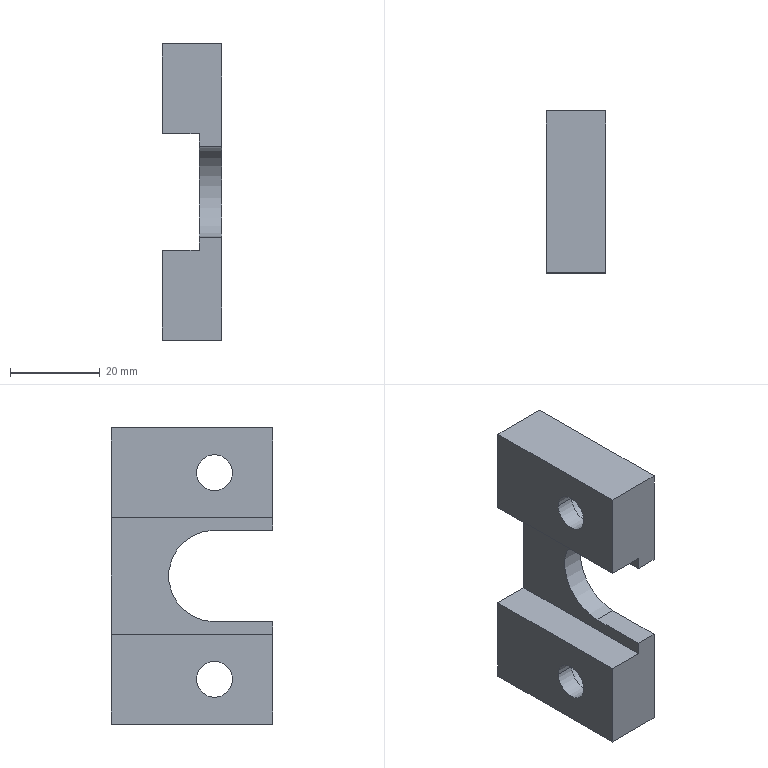Component | SolidWorks | ST60-12-1 | 1 solid | 24 faces | box 13.2 x 36 x 66 mm | volume 17942 mm3 | plane 15 | cylinder 9 | commonest cylinder face diameters 15 x4 8 x4 20.4 x1
build123d program:
from build123d import *

# Parameters (mm, degrees)
BOSS_EXTRUDE1_DEPTH                                = 46
CUT_EXTRUDE1_DEPTH                                 = 59.931
HOLE_SIZE_ACCORDING_TO_TYPE_1_OF_HEXAG_D           = 8
HOLE_SIZE_ACCORDING_TO_TYPE_1_OF_HEXAG_CBORE_D     = 15
HOLE_SIZE_ACCORDING_TO_TYPE_1_OF_HEXAG_CBORE_DEPTH = 9
SKETCH5_W                                          = 85.429
SKETCH5_H                                          = 31.164
CUT_EXTRUDE2_DEPTH                                 = 10


with BuildPart() as part:
    # Sketch1 → Boss-Extrude1 (new body)
    with BuildSketch(Plane.XY):
        Polygon((14.39, -6.081), (34.39, -6.081), (34.39, 7.119), (-31.61, 7.119), (-31.61, -6.081), (-11.61, -6.081), (-11.61, 2.119), (14.39, 2.119), align=None)
    extrude(amount=BOSS_EXTRUDE1_DEPTH)

    # Sketch2 → Cut-Extrude1 (cut, through all)
    with BuildSketch(Plane(origin=(0, 7.119, 0), x_dir=(1, 0, 0), z_dir=(0, 1, 0))):
        with BuildLine():
            Line((-8.81, -46), (-8.81, -23))
            ThreePointArc((-8.81, -23), (1.39, -12.8), (11.59, -23))
            Line((11.59, -23), (11.59, -46))
            ThreePointArc((11.59, -46), (1.39, -56.2), (-8.81, -46))
        make_face()
    extrude(amount=-CUT_EXTRUDE1_DEPTH, mode=Mode.SUBTRACT)

    # Hole Size _According to_ Type 1 of Hexag (through all)
    with Locations(Plane(origin=(0, 7.119, 0), x_dir=(1, 0, 0), z_dir=(0, 1, 0))):
        with Locations((-21.61, -23), (24.39, -23)):
            CounterBoreHole(HOLE_SIZE_ACCORDING_TO_TYPE_1_OF_HEXAG_D / 2, HOLE_SIZE_ACCORDING_TO_TYPE_1_OF_HEXAG_CBORE_D / 2, HOLE_SIZE_ACCORDING_TO_TYPE_1_OF_HEXAG_CBORE_DEPTH)

    # Sketch5 → Cut-Extrude2 (cut)
    with BuildSketch(Plane.XY.offset(46)):
        with Locations((-1.716, 2.752)):
            Rectangle(SKETCH5_W, SKETCH5_H)
    extrude(amount=-CUT_EXTRUDE2_DEPTH, mode=Mode.SUBTRACT)


solid = part.part

# Placed as in the assembly
solid = solid.moved(Location((158.075, 633.454, -1900.01), (90, 0, -90)))
STEP:
#1=CARTESIAN_POINT('',(6.149,24.329,-73.953));
#2=VERTEX_POINT('',#1);
#3=CARTESIAN_POINT('',(6.149,23.738,-73.953));
#4=VERTEX_POINT('',#3);
#5=CARTESIAN_POINT('',(6.149,24.034,-73.953));
#6=DIRECTION('',(1.,0.,-0.));
#7=DIRECTION('',(0.,-1.,0.));
#8=AXIS2_PLACEMENT_3D('',#5,#6,#7);
#9=CIRCLE('',#8,0.2953);
#10=EDGE_CURVE('',#2,#4,#9,.T.);
#11=ORIENTED_EDGE('',*,*,#10,.F.);
#12=CARTESIAN_POINT('',(6.504,24.329,-73.953));
#13=VERTEX_POINT('',#12);
#14=CARTESIAN_POINT('',(6.504,24.329,-73.953));
#15=DIRECTION('',(1.,0.,-0.));
#16=VECTOR('',#15,39.37);
#17=LINE('',#14,#16);
#18=EDGE_CURVE('',#2,#13,#17,.T.);
#19=ORIENTED_EDGE('',*,*,#18,.T.);
#20=CARTESIAN_POINT('',(6.504,23.738,-73.953));
#21=VERTEX_POINT('',#20);
#22=CARTESIAN_POINT('',(6.504,24.034,-73.953));
#23=DIRECTION('',(1.,0.,-0.));
#24=DIRECTION('',(0.,-1.,0.));
#25=AXIS2_PLACEMENT_3D('',#22,#23,#24);
#26=CIRCLE('',#25,0.2953);
#27=EDGE_CURVE('',#13,#21,#26,.T.);
#28=ORIENTED_EDGE('',*,*,#27,.T.);
#29=CARTESIAN_POINT('',(6.504,23.738,-73.953));
#30=DIRECTION('',(1.,0.,-0.));
#31=VECTOR('',#30,39.37);
#32=LINE('',#29,#31);
#33=EDGE_CURVE('',#4,#21,#32,.T.);
#34=ORIENTED_EDGE('',*,*,#33,.F.);
#35=EDGE_LOOP('',(#11,#19,#28,#34));
#36=FACE_OUTER_BOUND('',#35,.T.);
#37=CARTESIAN_POINT('',(6.504,24.034,-73.953));
#38=DIRECTION('',(1.,0.,-0.));
#39=DIRECTION('',(0.,-1.,0.));
#40=AXIS2_PLACEMENT_3D('',#37,#38,#39);
#41=CYLINDRICAL_SURFACE('',#40,0.2953);
#42=ADVANCED_FACE('',(#36),#41,.F.);
#43=CARTESIAN_POINT('',(5.984,24.191,-73.953));
#44=VERTEX_POINT('',#43);
#45=CARTESIAN_POINT('',(5.984,23.876,-73.953));
#46=VERTEX_POINT('',#45);
#47=CARTESIAN_POINT('',(5.984,24.034,-73.953));
#48=DIRECTION('',(1.,0.,-0.));
#49=DIRECTION('',(0.,-1.,0.));
#50=AXIS2_PLACEMENT_3D('',#47,#48,#49);
#51=CIRCLE('',#50,0.1575);
#52=EDGE_CURVE('',#44,#46,#51,.T.);
#53=ORIENTED_EDGE('',*,*,#52,.F.);
#54=CARTESIAN_POINT('',(6.149,24.191,-73.953));
#55=VERTEX_POINT('',#54);
#56=CARTESIAN_POINT('',(6.504,24.191,-73.953));
#57=DIRECTION('',(1.,0.,-0.));
#58=VECTOR('',#57,39.37);
#59=LINE('',#56,#58);
#60=EDGE_CURVE('',#44,#55,#59,.T.);
#61=ORIENTED_EDGE('',*,*,#60,.T.);
#62=CARTESIAN_POINT('',(6.149,23.876,-73.953));
#63=VERTEX_POINT('',#62);
#64=CARTESIAN_POINT('',(6.149,24.034,-73.953));
#65=DIRECTION('',(1.,0.,-0.));
#66=DIRECTION('',(0.,-1.,0.));
#67=AXIS2_PLACEMENT_3D('',#64,#65,#66);
#68=CIRCLE('',#67,0.1575);
#69=EDGE_CURVE('',#55,#63,#68,.T.);
#70=ORIENTED_EDGE('',*,*,#69,.T.);
#71=CARTESIAN_POINT('',(6.504,23.876,-73.953));
#72=DIRECTION('',(1.,0.,-0.));
#73=VECTOR('',#72,39.37);
#74=LINE('',#71,#73);
#75=EDGE_CURVE('',#46,#63,#74,.T.);
#76=ORIENTED_EDGE('',*,*,#75,.F.);
#77=EDGE_LOOP('',(#53,#61,#70,#76));
#78=FACE_OUTER_BOUND('',#77,.T.);
#79=CARTESIAN_POINT('',(6.504,24.034,-73.953));
#80=DIRECTION('',(1.,0.,-0.));
#81=DIRECTION('',(0.,-1.,0.));
#82=AXIS2_PLACEMENT_3D('',#79,#80,#81);
#83=CYLINDRICAL_SURFACE('',#82,0.1575);
#84=ADVANCED_FACE('',(#78),#83,.F.);
#85=CARTESIAN_POINT('',(6.149,24.329,-75.764));
#86=VERTEX_POINT('',#85);
#87=CARTESIAN_POINT('',(6.149,23.738,-75.764));
#88=VERTEX_POINT('',#87);
#89=CARTESIAN_POINT('',(6.149,24.034,-75.764));
#90=DIRECTION('',(1.,0.,-0.));
#91=DIRECTION('',(0.,-1.,0.));
#92=AXIS2_PLACEMENT_3D('',#89,#90,#91);
#93=CIRCLE('',#92,0.2953);
#94=EDGE_CURVE('',#86,#88,#93,.T.);
#95=ORIENTED_EDGE('',*,*,#94,.F.);
#96=CARTESIAN_POINT('',(6.504,24.329,-75.764));
#97=VERTEX_POINT('',#96);
#98=CARTESIAN_POINT('',(6.504,24.329,-75.764));
#99=DIRECTION('',(1.,0.,-0.));
#100=VECTOR('',#99,39.37);
#101=LINE('',#98,#100);
#102=EDGE_CURVE('',#86,#97,#101,.T.);
#103=ORIENTED_EDGE('',*,*,#102,.T.);
#104=CARTESIAN_POINT('',(6.504,23.738,-75.764));
#105=VERTEX_POINT('',#104);
#106=CARTESIAN_POINT('',(6.504,24.034,-75.764));
#107=DIRECTION('',(1.,0.,-0.));
#108=DIRECTION('',(0.,-1.,0.));
#109=AXIS2_PLACEMENT_3D('',#106,#107,#108);
#110=CIRCLE('',#109,0.2953);
#111=EDGE_CURVE('',#97,#105,#110,.T.);
#112=ORIENTED_EDGE('',*,*,#111,.T.);
#113=CARTESIAN_POINT('',(6.504,23.738,-75.764));
#114=DIRECTION('',(1.,0.,-0.));
#115=VECTOR('',#114,39.37);
#116=LINE('',#113,#115);
#117=EDGE_CURVE('',#88,#105,#116,.T.);
#118=ORIENTED_EDGE('',*,*,#117,.F.);
#119=EDGE_LOOP('',(#95,#103,#112,#118));
#120=FACE_OUTER_BOUND('',#119,.T.);
#121=CARTESIAN_POINT('',(6.504,24.034,-75.764));
#122=DIRECTION('',(1.,0.,-0.));
#123=DIRECTION('',(0.,-1.,0.));
#124=AXIS2_PLACEMENT_3D('',#121,#122,#123);
#125=CYLINDRICAL_SURFACE('',#124,0.2953);
#126=ADVANCED_FACE('',(#120),#125,.F.);
#127=CARTESIAN_POINT('',(5.984,24.191,-75.764));
#128=VERTEX_POINT('',#127);
#129=CARTESIAN_POINT('',(5.984,23.876,-75.764));
#130=VERTEX_POINT('',#129);
#131=CARTESIAN_POINT('',(5.984,24.034,-75.764));
#132=DIRECTION('',(1.,0.,-0.));
#133=DIRECTION('',(0.,-1.,0.));
#134=AXIS2_PLACEMENT_3D('',#131,#132,#133);
#135=CIRCLE('',#134,0.1575);
#136=EDGE_CURVE('',#128,#130,#135,.T.);
#137=ORIENTED_EDGE('',*,*,#136,.F.);
#138=CARTESIAN_POINT('',(6.149,24.191,-75.764));
#139=VERTEX_POINT('',#138);
#140=CARTESIAN_POINT('',(6.504,24.191,-75.764));
#141=DIRECTION('',(1.,0.,-0.));
#142=VECTOR('',#141,39.37);
#143=LINE('',#140,#142);
#144=EDGE_CURVE('',#128,#139,#143,.T.);
#145=ORIENTED_EDGE('',*,*,#144,.T.);
#146=CARTESIAN_POINT('',(6.149,23.876,-75.764));
#147=VERTEX_POINT('',#146);
#148=CARTESIAN_POINT('',(6.149,24.034,-75.764));
#149=DIRECTION('',(1.,0.,-0.));
#150=DIRECTION('',(0.,-1.,0.));
#151=AXIS2_PLACEMENT_3D('',#148,#149,#150);
#152=CIRCLE('',#151,0.1575);
#153=EDGE_CURVE('',#139,#147,#152,.T.);
#154=ORIENTED_EDGE('',*,*,#153,.T.);
#155=CARTESIAN_POINT('',(6.504,23.876,-75.764));
#156=DIRECTION('',(1.,0.,-0.));
#157=VECTOR('',#156,39.37);
#158=LINE('',#155,#157);
#159=EDGE_CURVE('',#130,#147,#158,.T.);
#160=ORIENTED_EDGE('',*,*,#159,.F.);
#161=EDGE_LOOP('',(#137,#145,#154,#160));
#162=FACE_OUTER_BOUND('',#161,.T.);
#163=CARTESIAN_POINT('',(6.504,24.034,-75.764));
#164=DIRECTION('',(1.,0.,-0.));
#165=DIRECTION('',(0.,-1.,0.));
#166=AXIS2_PLACEMENT_3D('',#163,#164,#165);
#167=CYLINDRICAL_SURFACE('',#166,0.1575);
#168=ADVANCED_FACE('',(#162),#167,.F.);
#169=CARTESIAN_POINT('',(6.504,23.522,-73.559));
#170=VERTEX_POINT('',#169);
#171=CARTESIAN_POINT('',(5.984,23.522,-73.559));
#172=VERTEX_POINT('',#171);
#173=CARTESIAN_POINT('',(6.504,23.522,-73.559));
#174=DIRECTION('',(-1.,-0.,0.));
#175=VECTOR('',#174,39.37);
#176=LINE('',#173,#175);
#177=EDGE_CURVE('',#170,#172,#176,.T.);
#178=ORIENTED_EDGE('',*,*,#177,.F.);
#179=CARTESIAN_POINT('',(6.504,24.939,-73.559));
#180=VERTEX_POINT('',#179);
#181=CARTESIAN_POINT('',(6.504,23.128,-73.559));
#182=DIRECTION('',(-0.,1.,0.));
#183=VECTOR('',#182,39.37);
#184=LINE('',#181,#183);
#185=EDGE_CURVE('',#170,#180,#184,.T.);
#186=ORIENTED_EDGE('',*,*,#185,.T.);
#187=CARTESIAN_POINT('',(5.984,24.939,-73.559));
#188=VERTEX_POINT('',#187);
#189=CARTESIAN_POINT('',(6.504,24.939,-73.559));
#190=DIRECTION('',(-1.,-0.,0.));
#191=VECTOR('',#190,39.37);
#192=LINE('',#189,#191);
#193=EDGE_CURVE('',#180,#188,#192,.T.);
#194=ORIENTED_EDGE('',*,*,#193,.T.);
#195=CARTESIAN_POINT('',(5.984,23.128,-73.559));
#196=DIRECTION('',(-0.,1.,0.));
#197=VECTOR('',#196,39.37);
#198=LINE('',#195,#197);
#199=EDGE_CURVE('',#172,#188,#198,.T.);
#200=ORIENTED_EDGE('',*,*,#199,.F.);
#201=EDGE_LOOP('',(#178,#186,#194,#200));
#202=FACE_OUTER_BOUND('',#201,.T.);
#203=CARTESIAN_POINT('',(6.504,23.128,-73.559));
#204=DIRECTION('',(-0.,0.,-1.));
#205=DIRECTION('',(-0.,1.,0.));
#206=AXIS2_PLACEMENT_3D('',#203,#204,#205);
#207=PLANE('',#206);
#208=ADVANCED_FACE('',(#202),#207,.F.);
#209=CARTESIAN_POINT('',(5.984,24.034,-73.953));
#210=DIRECTION('',(1.,0.,-0.));
#211=DIRECTION('',(0.,-1.,0.));
#212=AXIS2_PLACEMENT_3D('',#209,#210,#211);
#213=CIRCLE('',#212,0.1575);
#214=EDGE_CURVE('',#46,#44,#213,.T.);
#215=ORIENTED_EDGE('',*,*,#214,.T.);
#216=ORIENTED_EDGE('',*,*,#52,.T.);
#217=EDGE_LOOP('',(#215,#216));
#218=FACE_BOUND('',#217,.T.);
#219=CARTESIAN_POINT('',(5.984,23.522,-74.346));
#220=VERTEX_POINT('',#219);
#221=CARTESIAN_POINT('',(5.984,23.522,-73.559));
#222=DIRECTION('',(-0.,0.,-1.));
#223=VECTOR('',#222,39.37);
#224=LINE('',#221,#223);
#225=EDGE_CURVE('',#172,#220,#224,.T.);
#226=ORIENTED_EDGE('',*,*,#225,.F.);
#227=ORIENTED_EDGE('',*,*,#199,.T.);
#228=CARTESIAN_POINT('',(5.984,24.939,-74.346));
#229=VERTEX_POINT('',#228);
#230=CARTESIAN_POINT('',(5.984,24.939,-73.559));
#231=DIRECTION('',(-0.,0.,-1.));
#232=VECTOR('',#231,39.37);
#233=LINE('',#230,#232);
#234=EDGE_CURVE('',#188,#229,#233,.T.);
#235=ORIENTED_EDGE('',*,*,#234,.T.);
#236=CARTESIAN_POINT('',(5.984,23.128,-74.346));
#237=DIRECTION('',(-0.,1.,0.));
#238=VECTOR('',#237,39.37);
#239=LINE('',#236,#238);
#240=EDGE_CURVE('',#220,#229,#239,.T.);
#241=ORIENTED_EDGE('',*,*,#240,.F.);
#242=EDGE_LOOP('',(#226,#227,#235,#241));
#243=FACE_OUTER_BOUND('',#242,.T.);
#244=CARTESIAN_POINT('',(5.984,23.128,-73.559));
#245=DIRECTION('',(1.,0.,-0.));
#246=DIRECTION('',(0.,-1.,-0.));
#247=AXIS2_PLACEMENT_3D('',#244,#245,#246);
#248=PLANE('',#247);
#249=ADVANCED_FACE('',(#218,#243),#248,.F.);
#250=CARTESIAN_POINT('',(6.307,23.522,-74.346));
#251=VERTEX_POINT('',#250);
#252=CARTESIAN_POINT('',(5.984,23.522,-74.346));
#253=DIRECTION('',(1.,0.,-0.));
#254=VECTOR('',#253,39.37);
#255=LINE('',#252,#254);
#256=EDGE_CURVE('',#220,#251,#255,.T.);
#257=ORIENTED_EDGE('',*,*,#256,.F.);
#258=ORIENTED_EDGE('',*,*,#240,.T.);
#259=CARTESIAN_POINT('',(6.307,24.939,-74.346));
#260=VERTEX_POINT('',#259);
#261=CARTESIAN_POINT('',(5.984,24.939,-74.346));
#262=DIRECTION('',(1.,0.,-0.));
#263=VECTOR('',#262,39.37);
#264=LINE('',#261,#263);
#265=EDGE_CURVE('',#229,#260,#264,.T.);
#266=ORIENTED_EDGE('',*,*,#265,.T.);
#267=CARTESIAN_POINT('',(6.307,23.128,-74.346));
#268=DIRECTION('',(-0.,1.,0.));
#269=VECTOR('',#268,39.37);
#270=LINE('',#267,#269);
#271=EDGE_CURVE('',#251,#260,#270,.T.);
#272=ORIENTED_EDGE('',*,*,#271,.F.);
#273=EDGE_LOOP('',(#257,#258,#266,#272));
#274=FACE_OUTER_BOUND('',#273,.T.);
#275=CARTESIAN_POINT('',(5.984,23.128,-74.346));
#276=DIRECTION('',(0.,-0.,1.));
#277=DIRECTION('',(-1.,-0.,0.));
#278=AXIS2_PLACEMENT_3D('',#275,#276,#277);
#279=PLANE('',#278);
#280=ADVANCED_FACE('',(#274),#279,.F.);
#281=CARTESIAN_POINT('',(6.307,23.522,-74.457));
#282=VERTEX_POINT('',#281);
#283=CARTESIAN_POINT('',(6.307,23.522,-74.346));
#284=DIRECTION('',(-0.,0.,-1.));
#285=VECTOR('',#284,39.37);
#286=LINE('',#283,#285);
#287=EDGE_CURVE('',#251,#282,#286,.T.);
#288=ORIENTED_EDGE('',*,*,#287,.F.);
#289=ORIENTED_EDGE('',*,*,#271,.T.);
#290=CARTESIAN_POINT('',(6.307,24.939,-75.37));
#291=VERTEX_POINT('',#290);
#292=CARTESIAN_POINT('',(6.307,24.939,-74.346));
#293=DIRECTION('',(-0.,0.,-1.));
#294=VECTOR('',#293,39.37);
#295=LINE('',#292,#294);
#296=EDGE_CURVE('',#260,#291,#295,.T.);
#297=ORIENTED_EDGE('',*,*,#296,.T.);
#298=CARTESIAN_POINT('',(6.307,23.522,-75.37));
#299=VERTEX_POINT('',#298);
#300=CARTESIAN_POINT('',(6.307,23.128,-75.37));
#301=DIRECTION('',(-0.,1.,0.));
#302=VECTOR('',#301,39.37);
#303=LINE('',#300,#302);
#304=EDGE_CURVE('',#299,#291,#303,.T.);
#305=ORIENTED_EDGE('',*,*,#304,.F.);
#306=CARTESIAN_POINT('',(6.307,23.522,-75.26));
#307=VERTEX_POINT('',#306);
#308=CARTESIAN_POINT('',(6.307,23.522,-74.346));
#309=DIRECTION('',(-0.,0.,-1.));
#310=VECTOR('',#309,39.37);
#311=LINE('',#308,#310);
#312=EDGE_CURVE('',#307,#299,#311,.T.);
#313=ORIENTED_EDGE('',*,*,#312,.F.);
#314=CARTESIAN_POINT('',(6.307,24.034,-75.26));
#315=VERTEX_POINT('',#314);
#316=CARTESIAN_POINT('',(6.307,23.128,-75.26));
#317=DIRECTION('',(-0.,1.,0.));
#318=VECTOR('',#317,39.37);
#319=LINE('',#316,#318);
#320=EDGE_CURVE('',#307,#315,#319,.T.);
#321=ORIENTED_EDGE('',*,*,#320,.T.);
#322=CARTESIAN_POINT('',(6.307,24.034,-74.457));
#323=VERTEX_POINT('',#322);
#324=CARTESIAN_POINT('',(6.307,24.034,-74.858));
#325=DIRECTION('',(1.,0.,-0.));
#326=DIRECTION('',(0.,-1.,0.));
#327=AXIS2_PLACEMENT_3D('',#324,#325,#326);
#328=CIRCLE('',#327,0.4016);
#329=EDGE_CURVE('',#315,#323,#328,.T.);
#330=ORIENTED_EDGE('',*,*,#329,.T.);
#331=CARTESIAN_POINT('',(6.307,23.128,-74.457));
#332=DIRECTION('',(0.,-1.,-0.));
#333=VECTOR('',#332,39.37);
#334=LINE('',#331,#333);
#335=EDGE_CURVE('',#323,#282,#334,.T.);
#336=ORIENTED_EDGE('',*,*,#335,.T.);
#337=EDGE_LOOP('',(#288,#289,#297,#305,#313,#321,#330,#336));
#338=FACE_OUTER_BOUND('',#337,.T.);
#339=CARTESIAN_POINT('',(6.307,23.128,-74.346));
#340=DIRECTION('',(1.,0.,-0.));
#341=DIRECTION('',(0.,-1.,-0.));
#342=AXIS2_PLACEMENT_3D('',#339,#340,#341);
#343=PLANE('',#342);
#344=ADVANCED_FACE('',(#338),#343,.F.);
#345=CARTESIAN_POINT('',(5.984,23.522,-75.37));
#346=VERTEX_POINT('',#345);
#347=CARTESIAN_POINT('',(5.984,23.522,-75.37));
#348=DIRECTION('',(-1.,-0.,0.));
#349=VECTOR('',#348,39.37);
#350=LINE('',#347,#349);
#351=EDGE_CURVE('',#299,#346,#350,.T.);
#352=ORIENTED_EDGE('',*,*,#351,.F.);
#353=ORIENTED_EDGE('',*,*,#304,.T.);
#354=CARTESIAN_POINT('',(5.984,24.939,-75.37));
#355=VERTEX_POINT('',#354);
#356=CARTESIAN_POINT('',(5.984,24.939,-75.37));
#357=DIRECTION('',(-1.,-0.,0.));
#358=VECTOR('',#357,39.37);
#359=LINE('',#356,#358);
#360=EDGE_CURVE('',#291,#355,#359,.T.);
#361=ORIENTED_EDGE('',*,*,#360,.T.);
#362=CARTESIAN_POINT('',(5.984,23.128,-75.37));
#363=DIRECTION('',(-0.,1.,0.));
#364=VECTOR('',#363,39.37);
#365=LINE('',#362,#364);
#366=EDGE_CURVE('',#346,#355,#365,.T.);
#367=ORIENTED_EDGE('',*,*,#366,.F.);
#368=EDGE_LOOP('',(#352,#353,#361,#367));
#369=FACE_OUTER_BOUND('',#368,.T.);
#370=CARTESIAN_POINT('',(5.984,23.128,-75.37));
#371=DIRECTION('',(-0.,0.,-1.));
#372=DIRECTION('',(-0.,1.,0.));
#373=AXIS2_PLACEMENT_3D('',#370,#371,#372);
#374=PLANE('',#373);
#375=ADVANCED_FACE('',(#369),#374,.F.);
#376=CARTESIAN_POINT('',(5.984,24.034,-75.764));
#377=DIRECTION('',(1.,0.,-0.));
#378=DIRECTION('',(0.,-1.,0.));
#379=AXIS2_PLACEMENT_3D('',#376,#377,#378);
#380=CIRCLE('',#379,0.1575);
#381=EDGE_CURVE('',#130,#128,#380,.T.);
#382=ORIENTED_EDGE('',*,*,#381,.T.);
#383=ORIENTED_EDGE('',*,*,#136,.T.);
#384=EDGE_LOOP('',(#382,#383));
#385=FACE_BOUND('',#384,.T.);
#386=CARTESIAN_POINT('',(5.984,23.522,-76.157));
#387=VERTEX_POINT('',#386);
#388=CARTESIAN_POINT('',(5.984,23.522,-75.37));
#389=DIRECTION('',(-0.,0.,-1.));
#390=VECTOR('',#389,39.37);
#391=LINE('',#388,#390);
#392=EDGE_CURVE('',#346,#387,#391,.T.);
#393=ORIENTED_EDGE('',*,*,#392,.F.);
#394=ORIENTED_EDGE('',*,*,#366,.T.);
#395=CARTESIAN_POINT('',(5.984,24.939,-76.157));
#396=VERTEX_POINT('',#395);
#397=CARTESIAN_POINT('',(5.984,24.939,-75.37));
#398=DIRECTION('',(-0.,0.,-1.));
#399=VECTOR('',#398,39.37);
#400=LINE('',#397,#399);
#401=EDGE_CURVE('',#355,#396,#400,.T.);
#402=ORIENTED_EDGE('',*,*,#401,.T.);
#403=CARTESIAN_POINT('',(5.984,23.128,-76.157));
#404=DIRECTION('',(-0.,1.,0.));
#405=VECTOR('',#404,39.37);
#406=LINE('',#403,#405);
#407=EDGE_CURVE('',#387,#396,#406,.T.);
#408=ORIENTED_EDGE('',*,*,#407,.F.);
#409=EDGE_LOOP('',(#393,#394,#402,#408));
#410=FACE_OUTER_BOUND('',#409,.T.);
#411=CARTESIAN_POINT('',(5.984,23.128,-75.37));
#412=DIRECTION('',(1.,0.,-0.));
#413=DIRECTION('',(0.,-1.,-0.));
#414=AXIS2_PLACEMENT_3D('',#411,#412,#413);
#415=PLANE('',#414);
#416=ADVANCED_FACE('',(#385,#410),#415,.F.);
#417=CARTESIAN_POINT('',(6.504,23.522,-76.157));
#418=VERTEX_POINT('',#417);
#419=CARTESIAN_POINT('',(6.504,23.522,-76.157));
#420=DIRECTION('',(1.,0.,-0.));
#421=VECTOR('',#420,39.37);
#422=LINE('',#419,#421);
#423=EDGE_CURVE('',#387,#418,#422,.T.);
#424=ORIENTED_EDGE('',*,*,#423,.F.);
#425=ORIENTED_EDGE('',*,*,#407,.T.);
#426=CARTESIAN_POINT('',(6.504,24.939,-76.157));
#427=VERTEX_POINT('',#426);
#428=CARTESIAN_POINT('',(6.504,24.939,-76.157));
#429=DIRECTION('',(1.,0.,-0.));
#430=VECTOR('',#429,39.37);
#431=LINE('',#428,#430);
#432=EDGE_CURVE('',#396,#427,#431,.T.);
#433=ORIENTED_EDGE('',*,*,#432,.T.);
#434=CARTESIAN_POINT('',(6.504,23.128,-76.157));
#435=DIRECTION('',(-0.,1.,0.));
#436=VECTOR('',#435,39.37);
#437=LINE('',#434,#436);
#438=EDGE_CURVE('',#418,#427,#437,.T.);
#439=ORIENTED_EDGE('',*,*,#438,.F.);
#440=EDGE_LOOP('',(#424,#425,#433,#439));
#441=FACE_OUTER_BOUND('',#440,.T.);
#442=CARTESIAN_POINT('',(6.504,23.128,-76.157));
#443=DIRECTION('',(0.,-0.,1.));
#444=DIRECTION('',(0.,-1.,-0.));
#445=AXIS2_PLACEMENT_3D('',#442,#443,#444);
#446=PLANE('',#445);
#447=ADVANCED_FACE('',(#441),#446,.F.);
#448=CARTESIAN_POINT('',(6.504,24.034,-73.953));
#449=DIRECTION('',(1.,0.,-0.));
#450=DIRECTION('',(0.,-1.,0.));
#451=AXIS2_PLACEMENT_3D('',#448,#449,#450);
#452=CIRCLE('',#451,0.2953);
#453=EDGE_CURVE('',#21,#13,#452,.T.);
#454=ORIENTED_EDGE('',*,*,#453,.F.);
#455=ORIENTED_EDGE('',*,*,#27,.F.);
#456=EDGE_LOOP('',(#454,#455));
#457=FACE_BOUND('',#456,.T.);
#458=CARTESIAN_POINT('',(6.504,24.034,-75.764));
#459=DIRECTION('',(1.,0.,-0.));
#460=DIRECTION('',(0.,-1.,0.));
#461=AXIS2_PLACEMENT_3D('',#458,#459,#460);
#462=CIRCLE('',#461,0.2953);
#463=EDGE_CURVE('',#105,#97,#462,.T.);
#464=ORIENTED_EDGE('',*,*,#463,.F.);
#465=ORIENTED_EDGE('',*,*,#111,.F.);
#466=EDGE_LOOP('',(#464,#465));
#467=FACE_BOUND('',#466,.T.);
#468=CARTESIAN_POINT('',(6.504,23.522,-75.26));
#469=VERTEX_POINT('',#468);
#470=CARTESIAN_POINT('',(6.504,23.522,-73.559));
#471=DIRECTION('',(0.,-0.,1.));
#472=VECTOR('',#471,39.37);
#473=LINE('',#470,#472);
#474=EDGE_CURVE('',#418,#469,#473,.T.);
#475=ORIENTED_EDGE('',*,*,#474,.F.);
#476=ORIENTED_EDGE('',*,*,#438,.T.);
#477=CARTESIAN_POINT('',(6.504,24.939,-73.559));
#478=DIRECTION('',(0.,-0.,1.));
#479=VECTOR('',#478,39.37);
#480=LINE('',#477,#479);
#481=EDGE_CURVE('',#427,#180,#480,.T.);
#482=ORIENTED_EDGE('',*,*,#481,.T.);
#483=ORIENTED_EDGE('',*,*,#185,.F.);
#484=CARTESIAN_POINT('',(6.504,23.522,-74.457));
#485=VERTEX_POINT('',#484);
#486=CARTESIAN_POINT('',(6.504,23.522,-73.559));
#487=DIRECTION('',(0.,-0.,1.));
#488=VECTOR('',#487,39.37);
#489=LINE('',#486,#488);
#490=EDGE_CURVE('',#485,#170,#489,.T.);
#491=ORIENTED_EDGE('',*,*,#490,.F.);
#492=CARTESIAN_POINT('',(6.504,24.034,-74.457));
#493=VERTEX_POINT('',#492);
#494=CARTESIAN_POINT('',(6.504,23.128,-74.457));
#495=DIRECTION('',(0.,-1.,-0.));
#496=VECTOR('',#495,39.37);
#497=LINE('',#494,#496);
#498=EDGE_CURVE('',#493,#485,#497,.T.);
#499=ORIENTED_EDGE('',*,*,#498,.F.);
#500=CARTESIAN_POINT('',(6.504,24.034,-75.26));
#501=VERTEX_POINT('',#500);
#502=CARTESIAN_POINT('',(6.504,24.034,-74.858));
#503=DIRECTION('',(1.,0.,-0.));
#504=DIRECTION('',(0.,-1.,0.));
#505=AXIS2_PLACEMENT_3D('',#502,#503,#504);
#506=CIRCLE('',#505,0.4016);
#507=EDGE_CURVE('',#501,#493,#506,.T.);
#508=ORIENTED_EDGE('',*,*,#507,.F.);
#509=CARTESIAN_POINT('',(6.504,23.128,-75.26));
#510=DIRECTION('',(-0.,1.,0.));
#511=VECTOR('',#510,39.37);
#512=LINE('',#509,#511);
#513=EDGE_CURVE('',#469,#501,#512,.T.);
#514=ORIENTED_EDGE('',*,*,#513,.F.);
#515=EDGE_LOOP('',(#475,#476,#482,#483,#491,#499,#508,#514));
#516=FACE_OUTER_BOUND('',#515,.T.);
#517=CARTESIAN_POINT('',(6.504,23.128,-73.559));
#518=DIRECTION('',(-1.,-0.,0.));
#519=DIRECTION('',(-0.,1.,0.));
#520=AXIS2_PLACEMENT_3D('',#517,#518,#519);
#521=PLANE('',#520);
#522=ADVANCED_FACE('',(#457,#467,#516),#521,.F.);
#523=CARTESIAN_POINT('',(5.984,23.522,-74.457));
#524=DIRECTION('',(1.,0.,-0.));
#525=VECTOR('',#524,39.37);
#526=LINE('',#523,#525);
#527=EDGE_CURVE('',#282,#485,#526,.T.);
#528=ORIENTED_EDGE('',*,*,#527,.F.);
#529=ORIENTED_EDGE('',*,*,#335,.F.);
#530=CARTESIAN_POINT('',(5.984,24.034,-74.457));
#531=DIRECTION('',(1.,0.,-0.));
#532=VECTOR('',#531,39.37);
#533=LINE('',#530,#532);
#534=EDGE_CURVE('',#323,#493,#533,.T.);
#535=ORIENTED_EDGE('',*,*,#534,.T.);
#536=ORIENTED_EDGE('',*,*,#498,.T.);
#537=EDGE_LOOP('',(#528,#529,#535,#536));
#538=FACE_OUTER_BOUND('',#537,.T.);
#539=CARTESIAN_POINT('',(5.984,23.128,-74.457));
#540=DIRECTION('',(0.,-0.,1.));
#541=DIRECTION('',(0.,-1.,-0.));
#542=AXIS2_PLACEMENT_3D('',#539,#540,#541);
#543=PLANE('',#542);
#544=ADVANCED_FACE('',(#538),#543,.F.);
#545=CARTESIAN_POINT('',(5.984,23.522,-75.26));
#546=DIRECTION('',(-1.,-0.,0.));
#547=VECTOR('',#546,39.37);
#548=LINE('',#545,#547);
#549=EDGE_CURVE('',#469,#307,#548,.T.);
#550=ORIENTED_EDGE('',*,*,#549,.F.);
#551=ORIENTED_EDGE('',*,*,#513,.T.);
#552=CARTESIAN_POINT('',(5.984,24.034,-75.26));
#553=DIRECTION('',(1.,0.,-0.));
#554=VECTOR('',#553,39.37);
#555=LINE('',#552,#554);
#556=EDGE_CURVE('',#315,#501,#555,.T.);
#557=ORIENTED_EDGE('',*,*,#556,.F.);
#558=ORIENTED_EDGE('',*,*,#320,.F.);
#559=EDGE_LOOP('',(#550,#551,#557,#558));
#560=FACE_OUTER_BOUND('',#559,.T.);
#561=CARTESIAN_POINT('',(5.984,23.128,-75.26));
#562=DIRECTION('',(-0.,0.,-1.));
#563=DIRECTION('',(-0.,1.,0.));
#564=AXIS2_PLACEMENT_3D('',#561,#562,#563);
#565=PLANE('',#564);
#566=ADVANCED_FACE('',(#560),#565,.F.);
#567=ORIENTED_EDGE('',*,*,#193,.F.);
#568=ORIENTED_EDGE('',*,*,#481,.F.);
#569=ORIENTED_EDGE('',*,*,#432,.F.);
#570=ORIENTED_EDGE('',*,*,#401,.F.);
#571=ORIENTED_EDGE('',*,*,#360,.F.);
#572=ORIENTED_EDGE('',*,*,#296,.F.);
#573=ORIENTED_EDGE('',*,*,#265,.F.);
#574=ORIENTED_EDGE('',*,*,#234,.F.);
#575=EDGE_LOOP('',(#567,#568,#569,#570,#571,#572,#573,#574));
#576=FACE_OUTER_BOUND('',#575,.T.);
#577=CARTESIAN_POINT('',(6.223,24.939,-74.804));
#578=DIRECTION('',(0.,-1.,-0.));
#579=DIRECTION('',(-0.,0.,-1.));
#580=AXIS2_PLACEMENT_3D('',#577,#578,#579);
#581=PLANE('',#580);
#582=ADVANCED_FACE('',(#576),#581,.F.);
#583=ORIENTED_EDGE('',*,*,#556,.T.);
#584=ORIENTED_EDGE('',*,*,#507,.T.);
#585=ORIENTED_EDGE('',*,*,#534,.F.);
#586=ORIENTED_EDGE('',*,*,#329,.F.);
#587=EDGE_LOOP('',(#583,#584,#585,#586));
#588=FACE_OUTER_BOUND('',#587,.T.);
#589=CARTESIAN_POINT('',(5.984,24.034,-74.858));
#590=DIRECTION('',(1.,0.,-0.));
#591=DIRECTION('',(0.,-1.,0.));
#592=AXIS2_PLACEMENT_3D('',#589,#590,#591);
#593=CYLINDRICAL_SURFACE('',#592,0.4016);
#594=ADVANCED_FACE('',(#588),#593,.F.);
#595=ORIENTED_EDGE('',*,*,#144,.F.);
#596=ORIENTED_EDGE('',*,*,#381,.F.);
#597=ORIENTED_EDGE('',*,*,#159,.T.);
#598=CARTESIAN_POINT('',(6.149,24.034,-75.764));
#599=DIRECTION('',(1.,0.,-0.));
#600=DIRECTION('',(0.,-1.,0.));
#601=AXIS2_PLACEMENT_3D('',#598,#599,#600);
#602=CIRCLE('',#601,0.1575);
#603=EDGE_CURVE('',#147,#139,#602,.T.);
#604=ORIENTED_EDGE('',*,*,#603,.T.);
#605=EDGE_LOOP('',(#595,#596,#597,#604));
#606=FACE_OUTER_BOUND('',#605,.T.);
#607=CARTESIAN_POINT('',(6.504,24.034,-75.764));
#608=DIRECTION('',(1.,0.,-0.));
#609=DIRECTION('',(0.,-1.,0.));
#610=AXIS2_PLACEMENT_3D('',#607,#608,#609);
#611=CYLINDRICAL_SURFACE('',#610,0.1575);
#612=ADVANCED_FACE('',(#606),#611,.F.);
#613=ORIENTED_EDGE('',*,*,#603,.F.);
#614=ORIENTED_EDGE('',*,*,#153,.F.);
#615=EDGE_LOOP('',(#613,#614));
#616=FACE_BOUND('',#615,.T.);
#617=CARTESIAN_POINT('',(6.149,24.034,-75.764));
#618=DIRECTION('',(1.,0.,-0.));
#619=DIRECTION('',(0.,-1.,0.));
#620=AXIS2_PLACEMENT_3D('',#617,#618,#619);
#621=CIRCLE('',#620,0.2953);
#622=EDGE_CURVE('',#88,#86,#621,.T.);
#623=ORIENTED_EDGE('',*,*,#622,.T.);
#624=ORIENTED_EDGE('',*,*,#94,.T.);
#625=EDGE_LOOP('',(#623,#624));
#626=FACE_OUTER_BOUND('',#625,.T.);
#627=CARTESIAN_POINT('',(6.149,24.034,-75.921));
#628=DIRECTION('',(-1.,-0.,0.));
#629=DIRECTION('',(-0.,1.,0.));
#630=AXIS2_PLACEMENT_3D('',#627,#628,#629);
#631=PLANE('',#630);
#632=ADVANCED_FACE('',(#616,#626),#631,.F.);
#633=ORIENTED_EDGE('',*,*,#102,.F.);
#634=ORIENTED_EDGE('',*,*,#622,.F.);
#635=ORIENTED_EDGE('',*,*,#117,.T.);
#636=ORIENTED_EDGE('',*,*,#463,.T.);
#637=EDGE_LOOP('',(#633,#634,#635,#636));
#638=FACE_OUTER_BOUND('',#637,.T.);
#639=CARTESIAN_POINT('',(6.504,24.034,-75.764));
#640=DIRECTION('',(1.,0.,-0.));
#641=DIRECTION('',(0.,-1.,0.));
#642=AXIS2_PLACEMENT_3D('',#639,#640,#641);
#643=CYLINDRICAL_SURFACE('',#642,0.2953);
#644=ADVANCED_FACE('',(#638),#643,.F.);
#645=ORIENTED_EDGE('',*,*,#60,.F.);
#646=ORIENTED_EDGE('',*,*,#214,.F.);
#647=ORIENTED_EDGE('',*,*,#75,.T.);
#648=CARTESIAN_POINT('',(6.149,24.034,-73.953));
#649=DIRECTION('',(1.,0.,-0.));
#650=DIRECTION('',(0.,-1.,0.));
#651=AXIS2_PLACEMENT_3D('',#648,#649,#650);
#652=CIRCLE('',#651,0.1575);
#653=EDGE_CURVE('',#63,#55,#652,.T.);
#654=ORIENTED_EDGE('',*,*,#653,.T.);
#655=EDGE_LOOP('',(#645,#646,#647,#654));
#656=FACE_OUTER_BOUND('',#655,.T.);
#657=CARTESIAN_POINT('',(6.504,24.034,-73.953));
#658=DIRECTION('',(1.,0.,-0.));
#659=DIRECTION('',(0.,-1.,0.));
#660=AXIS2_PLACEMENT_3D('',#657,#658,#659);
#661=CYLINDRICAL_SURFACE('',#660,0.1575);
#662=ADVANCED_FACE('',(#656),#661,.F.);
#663=ORIENTED_EDGE('',*,*,#653,.F.);
#664=ORIENTED_EDGE('',*,*,#69,.F.);
#665=EDGE_LOOP('',(#663,#664));
#666=FACE_BOUND('',#665,.T.);
#667=CARTESIAN_POINT('',(6.149,24.034,-73.953));
#668=DIRECTION('',(1.,0.,-0.));
#669=DIRECTION('',(0.,-1.,0.));
#670=AXIS2_PLACEMENT_3D('',#667,#668,#669);
#671=CIRCLE('',#670,0.2953);
#672=EDGE_CURVE('',#4,#2,#671,.T.);
#673=ORIENTED_EDGE('',*,*,#672,.T.);
#674=ORIENTED_EDGE('',*,*,#10,.T.);
#675=EDGE_LOOP('',(#673,#674));
#676=FACE_OUTER_BOUND('',#675,.T.);
#677=CARTESIAN_POINT('',(6.149,24.034,-74.11));
#678=DIRECTION('',(-1.,-0.,0.));
#679=DIRECTION('',(-0.,1.,0.));
#680=AXIS2_PLACEMENT_3D('',#677,#678,#679);
#681=PLANE('',#680);
#682=ADVANCED_FACE('',(#666,#676),#681,.F.);
#683=ORIENTED_EDGE('',*,*,#18,.F.);
#684=ORIENTED_EDGE('',*,*,#672,.F.);
#685=ORIENTED_EDGE('',*,*,#33,.T.);
#686=ORIENTED_EDGE('',*,*,#453,.T.);
#687=EDGE_LOOP('',(#683,#684,#685,#686));
#688=FACE_OUTER_BOUND('',#687,.T.);
#689=CARTESIAN_POINT('',(6.504,24.034,-73.953));
#690=DIRECTION('',(1.,0.,-0.));
#691=DIRECTION('',(0.,-1.,0.));
#692=AXIS2_PLACEMENT_3D('',#689,#690,#691);
#693=CYLINDRICAL_SURFACE('',#692,0.2953);
#694=ADVANCED_FACE('',(#688),#693,.F.);
#695=ORIENTED_EDGE('',*,*,#312,.T.);
#696=ORIENTED_EDGE('',*,*,#351,.T.);
#697=ORIENTED_EDGE('',*,*,#392,.T.);
#698=ORIENTED_EDGE('',*,*,#423,.T.);
#699=ORIENTED_EDGE('',*,*,#474,.T.);
#700=ORIENTED_EDGE('',*,*,#549,.T.);
#701=EDGE_LOOP('',(#695,#696,#697,#698,#699,#700));
#702=FACE_OUTER_BOUND('',#701,.T.);
#703=CARTESIAN_POINT('',(6.223,23.522,-74.804));
#704=DIRECTION('',(0.,-1.,-0.));
#705=DIRECTION('',(-0.,0.,-1.));
#706=AXIS2_PLACEMENT_3D('',#703,#704,#705);
#707=PLANE('',#706);
#708=ADVANCED_FACE('',(#702),#707,.T.);
#709=ORIENTED_EDGE('',*,*,#177,.T.);
#710=ORIENTED_EDGE('',*,*,#225,.T.);
#711=ORIENTED_EDGE('',*,*,#256,.T.);
#712=ORIENTED_EDGE('',*,*,#287,.T.);
#713=ORIENTED_EDGE('',*,*,#527,.T.);
#714=ORIENTED_EDGE('',*,*,#490,.T.);
#715=EDGE_LOOP('',(#709,#710,#711,#712,#713,#714));
#716=FACE_OUTER_BOUND('',#715,.T.);
#717=CARTESIAN_POINT('',(6.223,23.522,-74.804));
#718=DIRECTION('',(0.,-1.,-0.));
#719=DIRECTION('',(-0.,0.,-1.));
#720=AXIS2_PLACEMENT_3D('',#717,#718,#719);
#721=PLANE('',#720);
#722=ADVANCED_FACE('',(#716),#721,.T.);
#723=CLOSED_SHELL('',(#42,#84,#126,#168,#208,#249,#280,#344,#375,#416,#447,#522,#544,#566,#582,#594,#612,#632,#644,#662,#682,#694,#708,#722));
#724=MANIFOLD_SOLID_BREP('',#723);
#725=CARTESIAN_POINT('',(0.,0.,0.));
#726=DIRECTION('',(0.,0.,1.));
#727=DIRECTION('',(1.,0.,0.));
#728=AXIS2_PLACEMENT_3D('',#725,#726,#727);
#729=(LENGTH_UNIT()NAMED_UNIT(*)SI_UNIT($,.METRE.));
#730=LENGTH_MEASURE_WITH_UNIT(LENGTH_MEASURE(0.0254),#729);
#731=DIMENSIONAL_EXPONENTS(1.,0.,0.,0.,0.,0.,0.);
#732=(CONVERSION_BASED_UNIT('',#730)LENGTH_UNIT()NAMED_UNIT(#731));
#733=UNCERTAINTY_MEASURE_WITH_UNIT(LENGTH_MEASURE(0.00001),#732,'','');
#734=(NAMED_UNIT(*)PLANE_ANGLE_UNIT()SI_UNIT($,.RADIAN.));
#735=(NAMED_UNIT(*)SI_UNIT($,.STERADIAN.)SOLID_ANGLE_UNIT());
#736=(GEOMETRIC_REPRESENTATION_CONTEXT(3)GLOBAL_UNCERTAINTY_ASSIGNED_CONTEXT((#733))GLOBAL_UNIT_ASSIGNED_CONTEXT((#732,#734,#735))REPRESENTATION_CONTEXT('',''));
#737=ADVANCED_BREP_SHAPE_REPRESENTATION('',(#724,#728),#736);
#738=COLOUR_RGB('',0.7922,0.8196,0.9333);
#739=FILL_AREA_STYLE_COLOUR('',#738);
#740=FILL_AREA_STYLE('',(#739));
#741=SURFACE_STYLE_FILL_AREA(#740);
#742=SURFACE_SIDE_STYLE('',(#741));
#743=SURFACE_STYLE_USAGE(.BOTH.,#742);
#744=PRESENTATION_STYLE_ASSIGNMENT((#743));
#745=STYLED_ITEM('',(#744),#724);
#746=(LENGTH_UNIT()NAMED_UNIT(*)SI_UNIT($,.METRE.));
#747=LENGTH_MEASURE_WITH_UNIT(LENGTH_MEASURE(0.0254),#746);
#748=DIMENSIONAL_EXPONENTS(1.,0.,0.,0.,0.,0.,0.);
#749=(CONVERSION_BASED_UNIT('',#747)LENGTH_UNIT()NAMED_UNIT(#748));
#750=UNCERTAINTY_MEASURE_WITH_UNIT(LENGTH_MEASURE(0.00001),#749,'','');
#751=(NAMED_UNIT(*)PLANE_ANGLE_UNIT()SI_UNIT($,.RADIAN.));
#752=(NAMED_UNIT(*)SI_UNIT($,.STERADIAN.)SOLID_ANGLE_UNIT());
#753=(GEOMETRIC_REPRESENTATION_CONTEXT(3)GLOBAL_UNCERTAINTY_ASSIGNED_CONTEXT((#750))GLOBAL_UNIT_ASSIGNED_CONTEXT((#749,#751,#752))REPRESENTATION_CONTEXT('',''));
#754=MECHANICAL_DESIGN_GEOMETRIC_PRESENTATION_REPRESENTATION('',(#745),#753);
#755=PRESENTATION_LAYER_ASSIGNMENT('','',(#745));